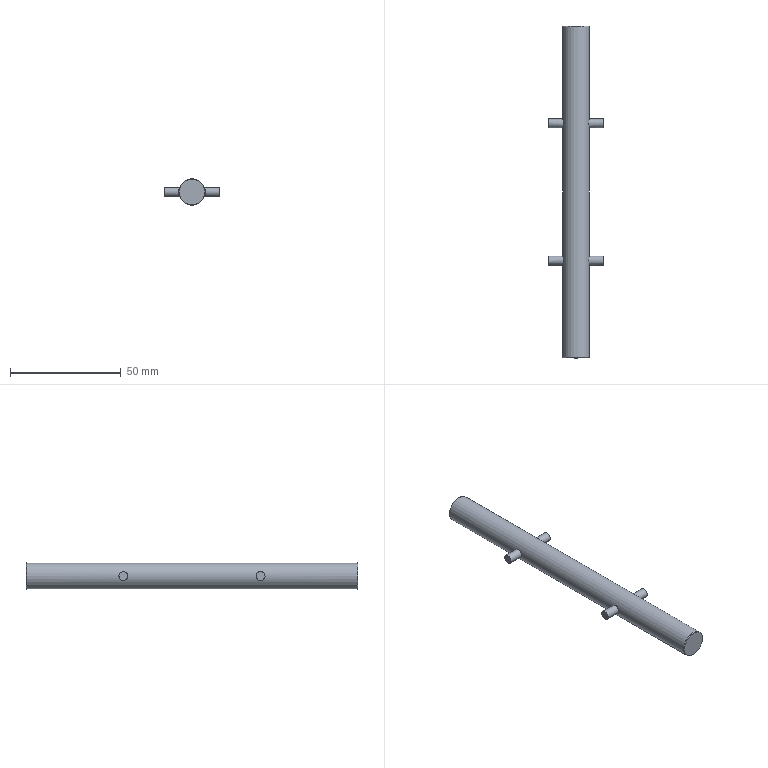Component | NX | SMALL_PULLEY_SHAFT | 1 solid | 13 faces | volume 17293 mm3 | plane 6 | cylinder 5 | cone 2 | commonest cylinder face diameters 4 x4 12 x1